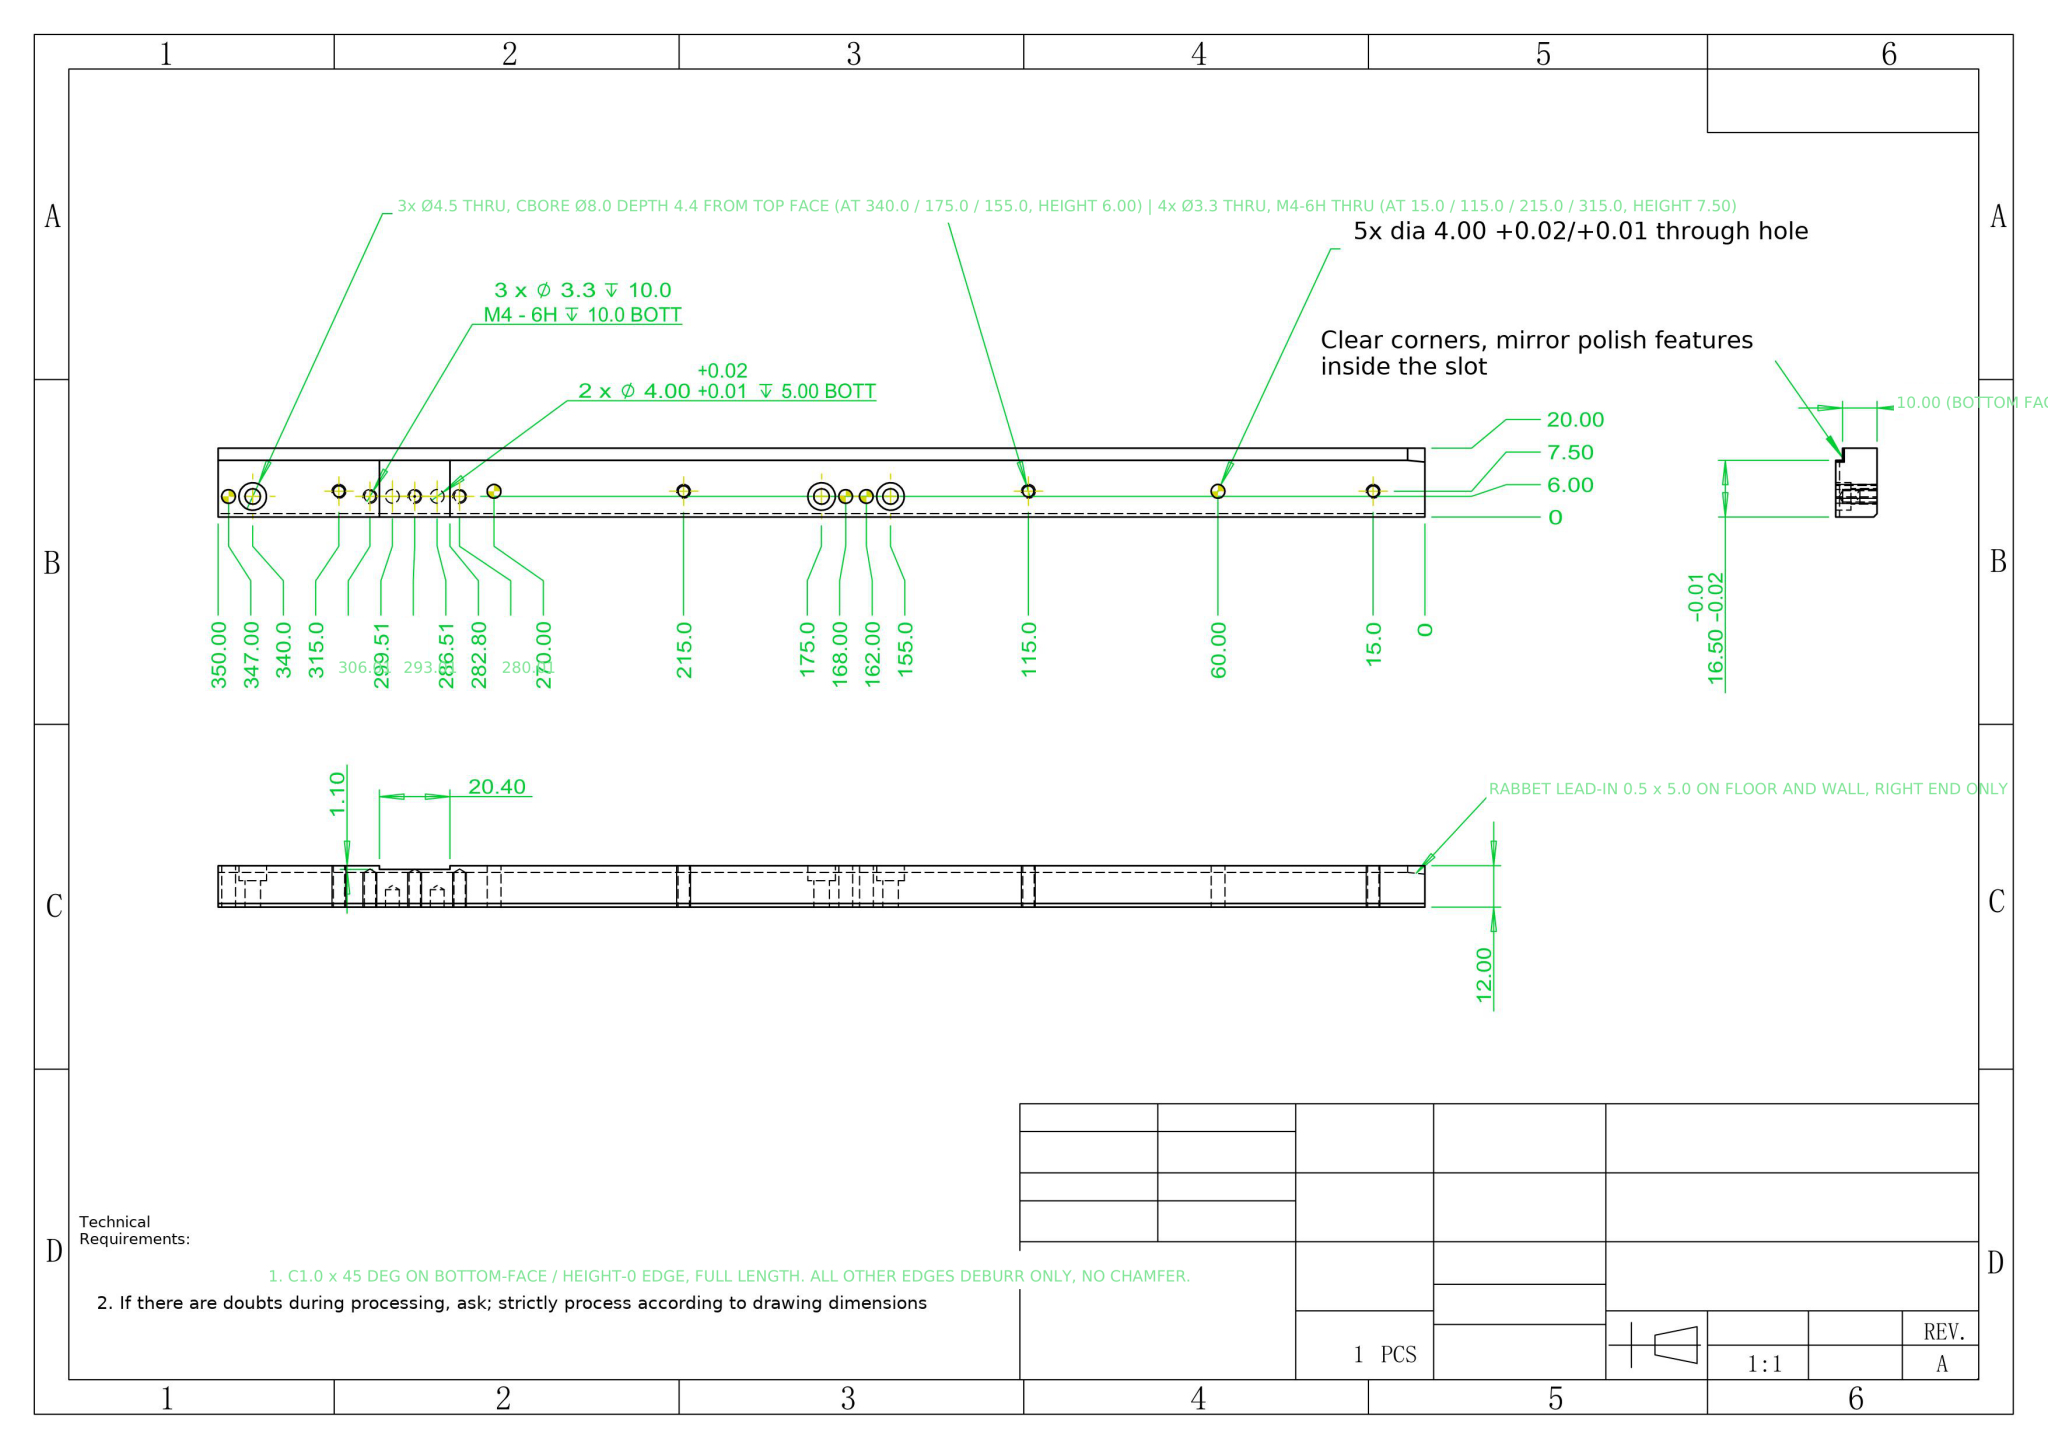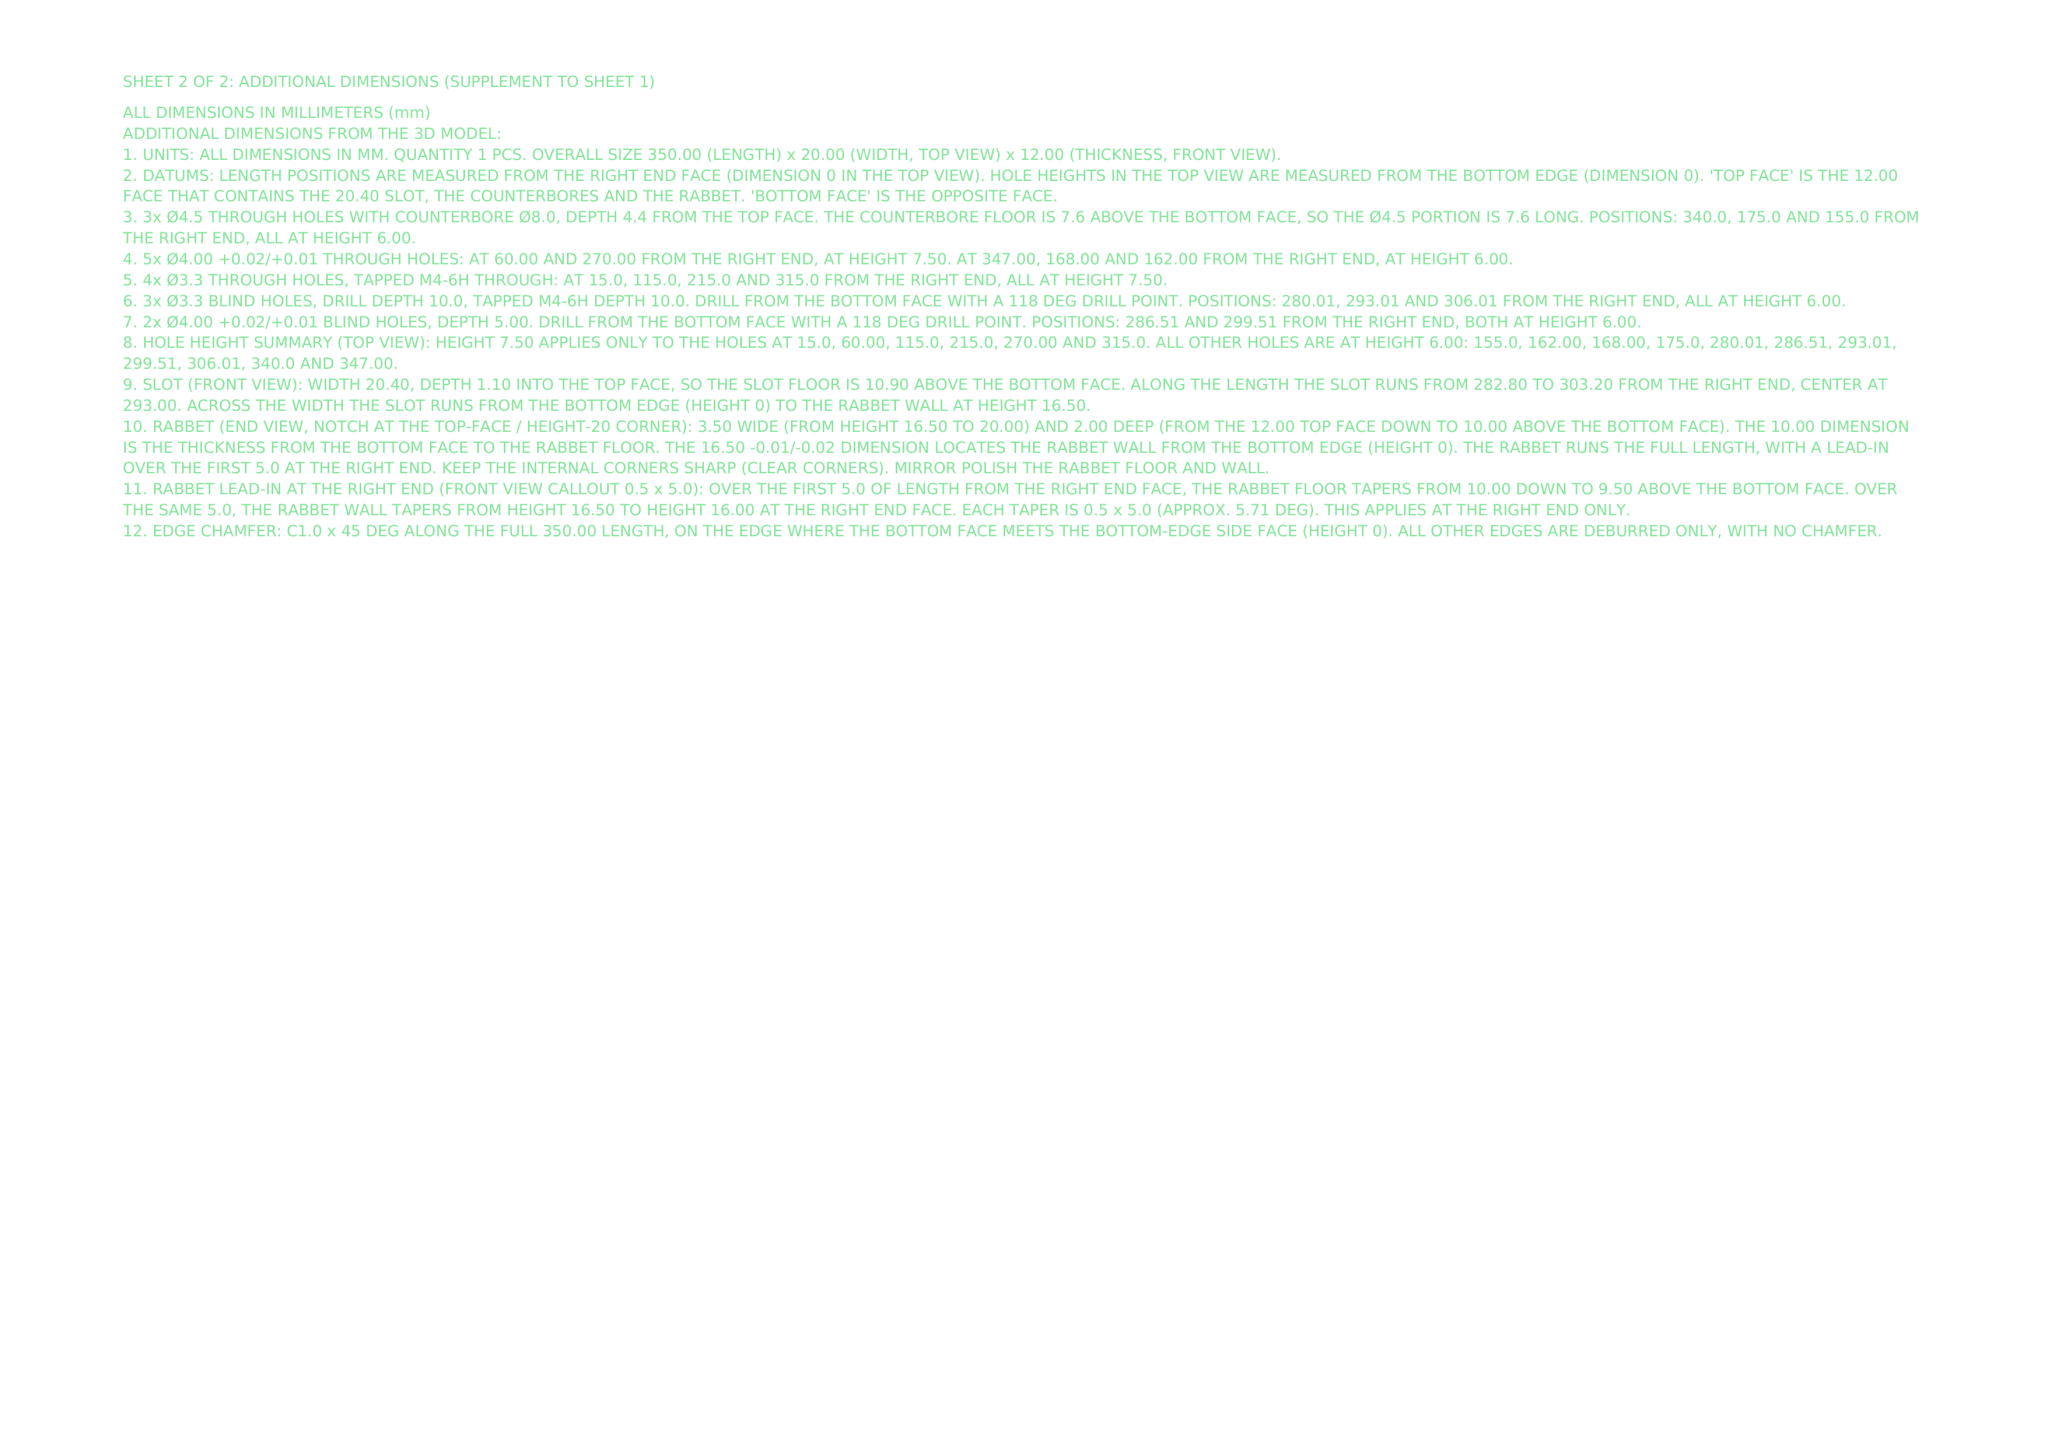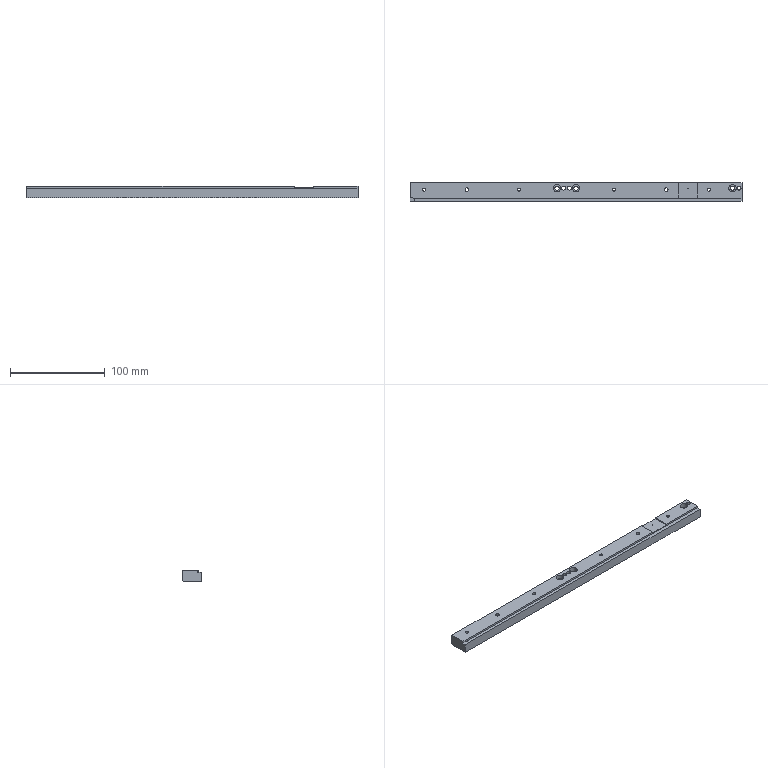Part | NX | mm | 1 solid | 68 faces | box 350 x 20 x 12 mm | volume 78406 mm3 | cylinder 40 | plane 18 | cone 10 | commonest cylinder face diameters 4 x14 3.3 x14 8 x6 4.5 x6